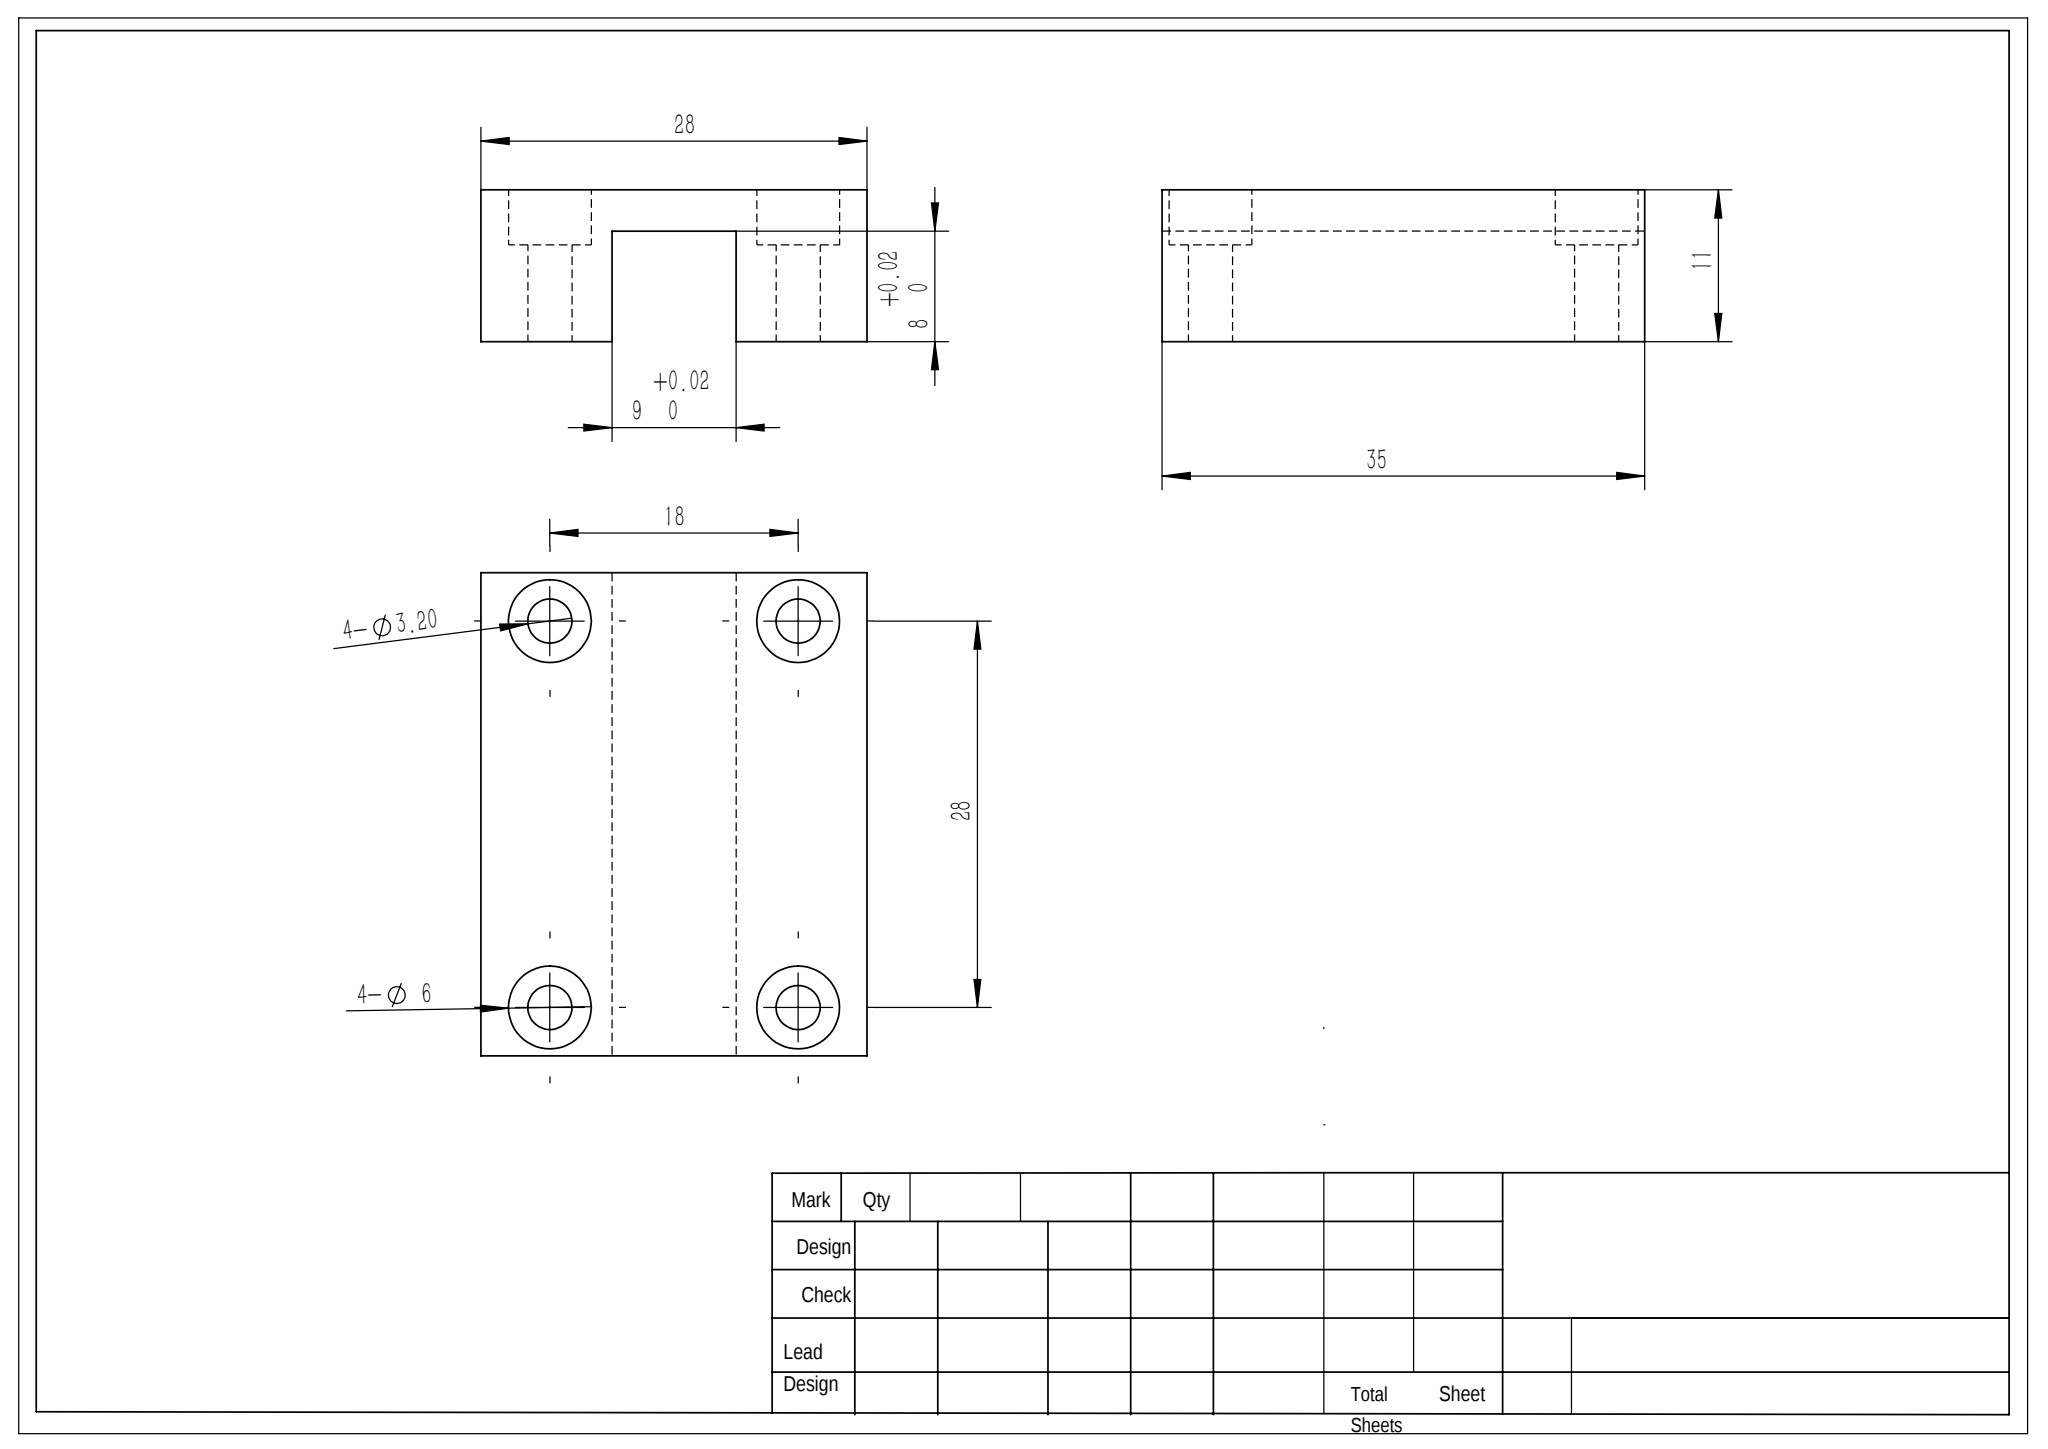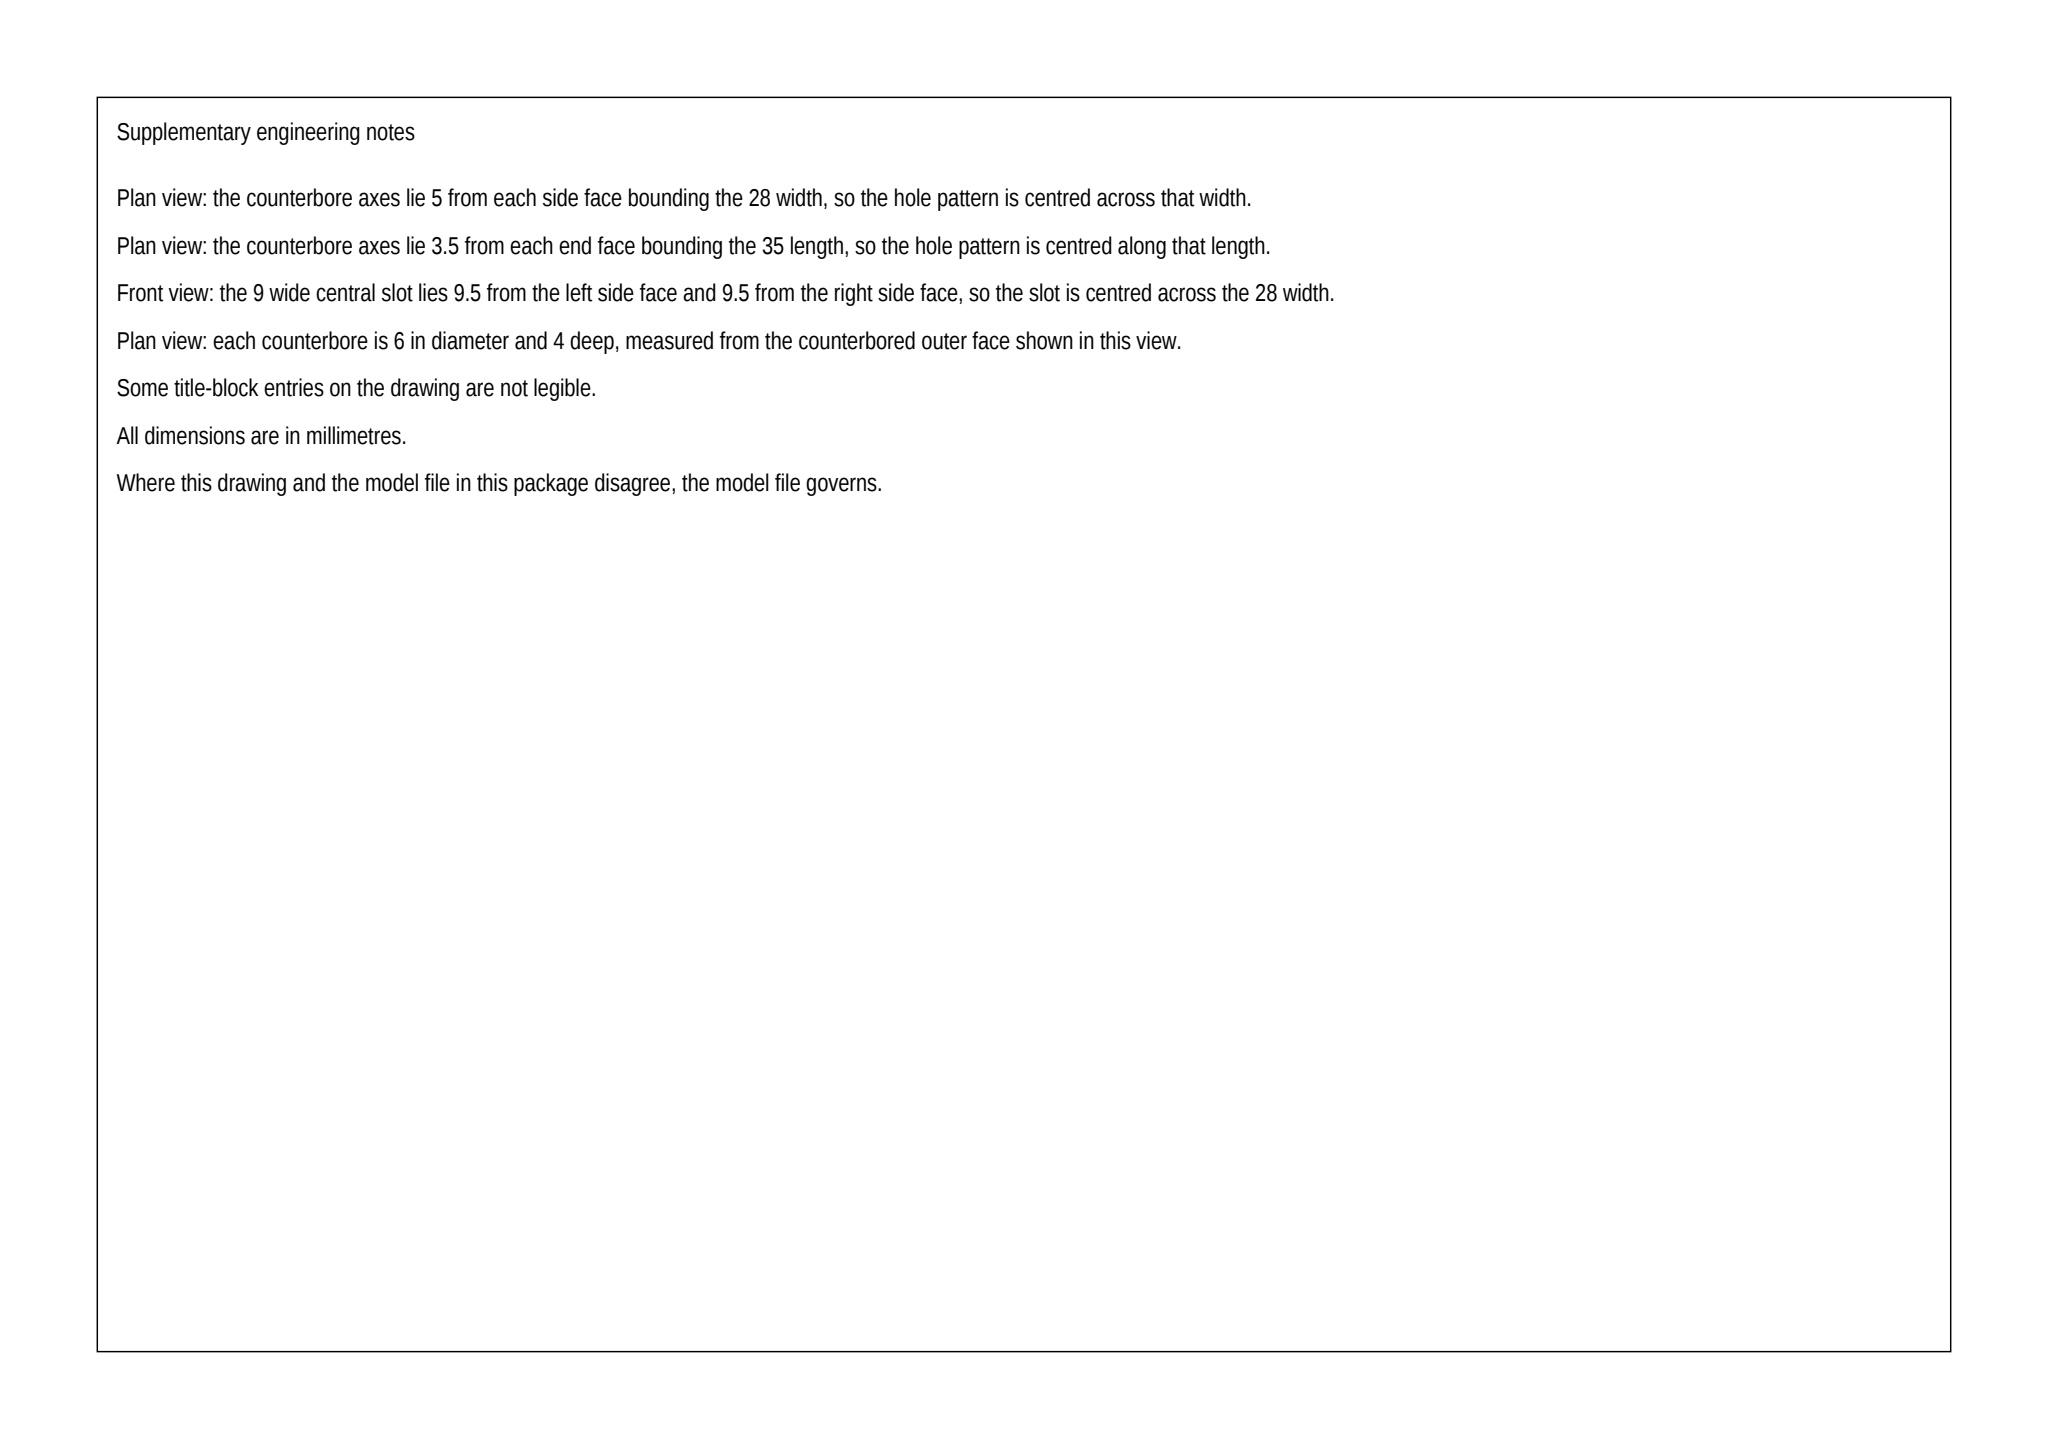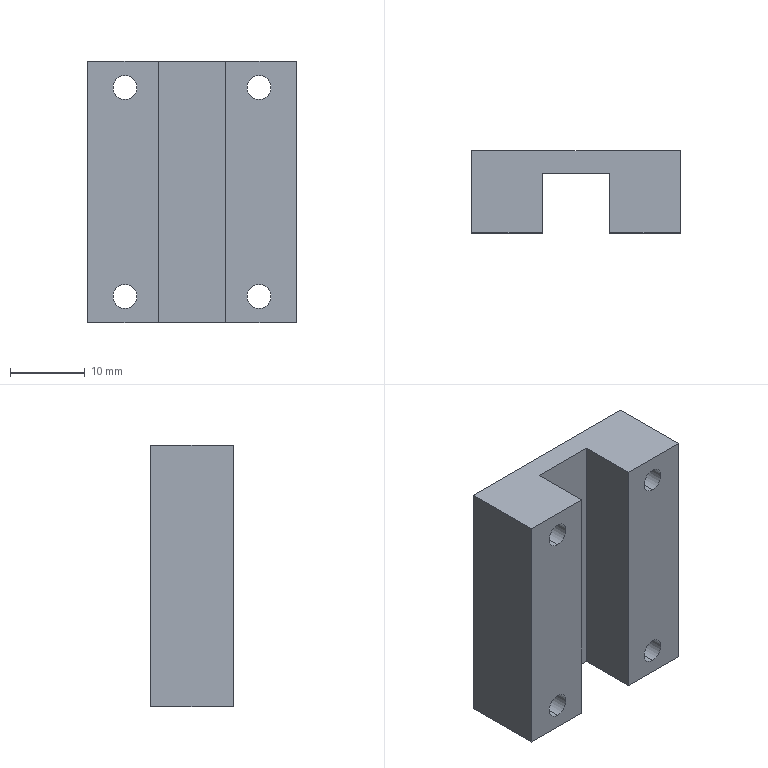Part | SolidWorks | mm | 1 solid | 30 faces | box 28 x 11 x 35 mm | volume 7582 mm3 | cylinder 16 | plane 14 | commonest cylinder face diameters 6 x8 3.2 x8
Drawing notes:
Ø6 C'BORE DP 4, 4 PLCS | from the solid: cyl dia 6.0 axis y length 4.0 (y 7.0 to 11.0), 4 locations
SHOULDER 9.5 WIDE EA SIDE OF 9 BOSS (28 OAL) | from the solid: x planes 0/9.5/18.5/28; boss 9 wide, flanges 9.5
4-Ø3.20 HOLE CL 5 FROM EA SIDE EDGE (18 APART) | from the solid: Ø3.2 holes at x=5.0 and x=23.0, bbox x=28
4-Ø3.20 HOLE CL 3.5 FROM EA END EDGE (28 APART) | from the solid: Ø3.2 holes at z=3.5 and z=31.5, bbox z=35
build123d program:
from build123d import *

# Parameters (mm, degrees)
BOSS_EXTRUDE1_DEPTH                           = 35
COUNTERBORE_FOR_M3_HEX_HEAD_BOLT1_D           = 3.2
COUNTERBORE_FOR_M3_HEX_HEAD_BOLT1_CBORE_D     = 6
COUNTERBORE_FOR_M3_HEX_HEAD_BOLT1_CBORE_DEPTH = 4


with BuildPart() as part:
    # Sketch1 → Boss-Extrude1 (new body)
    with BuildSketch(Plane.XY):
        Polygon((-15.426, 9.428), (12.574, 9.428), (12.574, -1.572), (3.074, -1.572), (3.074, 6.428), (-5.926, 6.428), (-5.926, -1.572), (-15.426, -1.572), align=None)
    extrude(amount=BOSS_EXTRUDE1_DEPTH)

    # Counterbore for M3 Hex Head Bolt1 (through all)
    with Locations(Plane(origin=(0, 9.428, 0), x_dir=(1, 0, 0), z_dir=(0, 1, 0))):
        with Locations((7.574, -31.5), (-10.426, -31.5), (-10.426, -3.5), (7.574, -3.5)):
            CounterBoreHole(COUNTERBORE_FOR_M3_HEX_HEAD_BOLT1_D / 2, COUNTERBORE_FOR_M3_HEX_HEAD_BOLT1_CBORE_D / 2, COUNTERBORE_FOR_M3_HEX_HEAD_BOLT1_CBORE_DEPTH)


solid = part.part